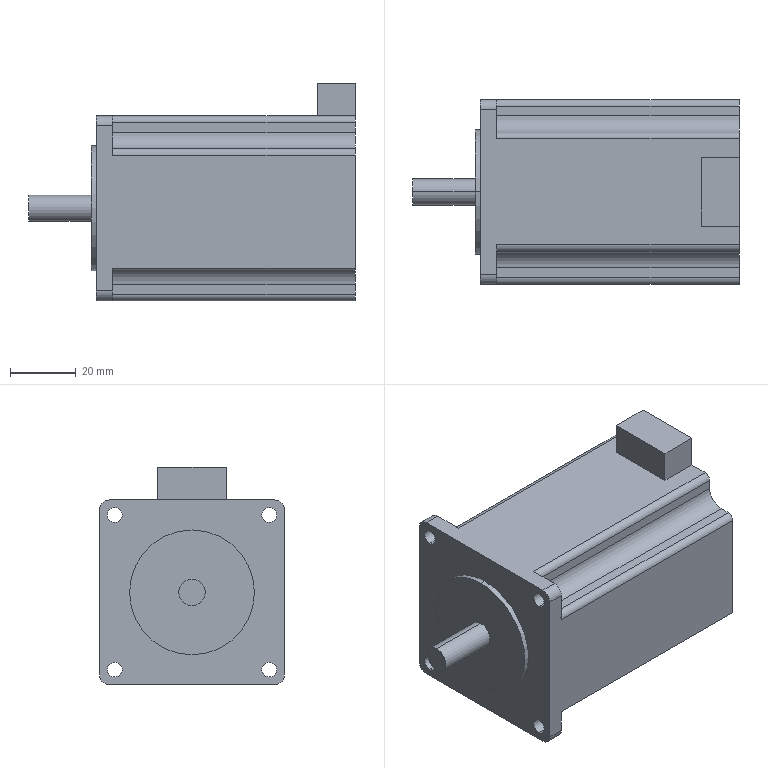Component | SolidWorks | Motor-57-1 | 1 solid | 51 faces | box 99.6 x 56.4 x 66.4 mm | volume 227698 mm3 | cylinder 27 | plane 24 | commonest cylinder face diameters 4.5 x8 4 x7 10 x4 6 x4 8 x2 38.1 x2
build123d program:
from build123d import *

# Parameters (mm, degrees)
SKETCH1_W            = 56.4
SKETCH1_H            = 56.4
BOSS_EXTRUDE1_DEPTH  = 79
SKETCH2_R            = 2.25
CUT_EXTRUDE1_DEPTH   = 113.263
LPATTERN1_COUNT      = 2
LPATTERN1_PITCH      = 47.14
LPATTERN1_COUNT_DIR2 = 2
LPATTERN1_PITCH_DIR2 = 47.14
SKETCH3_W            = 10
SKETCH3_H            = 10
CUT_EXTRUDE2_DEPTH   = 74
SKETCH4_R            = 19.05
BOSS_EXTRUDE2_DEPTH  = 1.6
SKETCH5_R            = 4
BOSS_EXTRUDE3_DEPTH  = 19
CIRPATTERN1_COUNT    = 4
FILLET1_R            = 5
FILLET2_R            = 2
SKETCH6_W            = 10
SKETCH6_H            = 21
BOSS_EXTRUDE4_DEPTH  = 11.6
FILLET3_R            = 3


with BuildPart() as part:
    # Sketch1 → Boss-Extrude1 (new body)
    with BuildSketch(Plane.XY):
        with Locations((28.2, -28.2)):
            Rectangle(SKETCH1_W, SKETCH1_H)
    extrude(amount=BOSS_EXTRUDE1_DEPTH)

    # Sketch2 → Cut-Extrude1 (cut, through all)
    with BuildSketch(Plane(origin=(0, 0, 0), x_dir=(-1, 0, 0), z_dir=(0, 0, -1))):
        with Locations((-51.77, -4.63)):
            Circle(SKETCH2_R)
    cut_extrude1 = extrude(amount=-CUT_EXTRUDE1_DEPTH, mode=Mode.SUBTRACT)

    # LPattern1: Cut-Extrude1 2 × 2
    with Locations(*[(-i * LPATTERN1_PITCH, -j * LPATTERN1_PITCH_DIR2, 0) for i in range(LPATTERN1_COUNT) for j in range(LPATTERN1_COUNT_DIR2) if (i, j) != (0, 0)]):
        add(cut_extrude1, mode=Mode.SUBTRACT)

    # Sketch3 → Cut-Extrude2 (cut)
    with BuildSketch(Plane(origin=(0, 0, 0), x_dir=(-1, 0, 0), z_dir=(0, 0, -1))):
        with Locations((-51.4, -5)):
            Rectangle(SKETCH3_W, SKETCH3_H)
    cut_extrude2 = extrude(amount=-CUT_EXTRUDE2_DEPTH, mode=Mode.SUBTRACT)

    # Sketch4 → Boss-Extrude2 (add)
    with BuildSketch(Plane.XY.offset(79)):
        with Locations((28.2, -28.2)):
            Circle(SKETCH4_R)
    extrude(amount=BOSS_EXTRUDE2_DEPTH)

    # Sketch5 → Boss-Extrude3 (add)
    with BuildSketch(Plane.XY.offset(80.6)):
        with Locations((28.2, -28.2)):
            Circle(SKETCH5_R)
    extrude(amount=BOSS_EXTRUDE3_DEPTH)

    # CirPattern1: Cut-Extrude2 ×4 about axis
    cirpattern1_axis = Axis((28.2, -28.2, 0), (0, 0, 1))
    for i in range(1, CIRPATTERN1_COUNT):
        add(cut_extrude2.rotate(cirpattern1_axis, i * 360 / CIRPATTERN1_COUNT), mode=Mode.SUBTRACT)

    # Fillet1
    fillet1_edges = [part.edges().sort_by_distance(p)[0] for p in [
        (46.4, -10, 37),
        (46.4, -46.4, 37),
        (10, -46.4, 37),
        (10, -10, 37),
    ]]
    fillet(fillet1_edges, radius=FILLET1_R)

    # Fillet2
    fillet2_edges = [part.edges().sort_by_distance(p)[0] for p in [
        (56.4, -10, 37),
        (46.4, 0, 37),
        (46.4, -56.4, 37),
        (56.4, -46.4, 37),
        (0, -46.4, 37),
        (10, 0, 37),
        (0, -10, 37),
    ]]
    fillet(fillet2_edges, radius=FILLET2_R)

    # Sketch6 → Boss-Extrude4 (add)
    with BuildSketch(Plane(origin=(0, 0, 0), x_dir=(-1, 0, 0), z_dir=(0, 0, -1))):
        with Locations((-61.4, -28.2)):
            Rectangle(SKETCH6_W, SKETCH6_H)
    extrude(amount=-BOSS_EXTRUDE4_DEPTH)

    # Fillet3
    fillet3_edges = [part.edges().sort_by_distance(p)[0] for p in [
        (0, 0, 76.5),
        (56.4, 0, 76.5),
        (56.4, -56.4, 76.5),
        (0, -56.4, 76.5),
    ]]
    fillet(fillet3_edges, radius=FILLET3_R)


solid = part.part

# Placed as in the assembly
solid = solid.moved(Location((183.478, 48.145, -24.649), (0, -90, 0)))